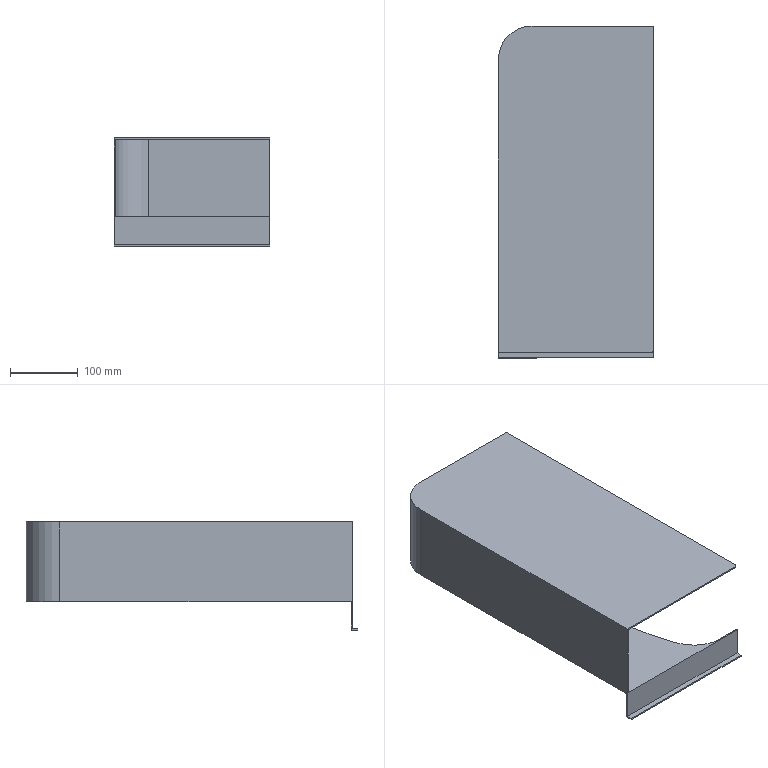Component | SolidWorks | AA-1_B-1 | 1 solid | 22 faces | box 230 x 491 x 160 mm | volume 563290 mm3 | plane 15 | cylinder 7 | commonest cylinder face diameters 120 x2 10 x2 100 x1 96 x1 948.312 x1
build123d program:
from build123d import *

# Parameters (mm, degrees)
SKETCH1_W           = 118
SKETCH1_H           = 483
BOSS_EXTRUDE1_DEPTH = 85
FILLET3_R           = 50
SHELL1_T            = -2
SKETCH3_W           = 170
SKETCH3_H           = 2
BOSS_EXTRUDE3_DEPTH = 40
SKETCH4_W           = 2
SKETCH4_H           = 170
BOSS_EXTRUDE4_DEPTH = 10
BOSS_EXTRUDE7_DEPTH = 30
BOSS_EXTRUDE8_DEPTH = 30
CUT_EXTRUDE7_DEPTH  = 2
CUT_EXTRUDE8_DEPTH  = 2
FILLET2_R           = 5
FILLET4_R           = 5


with BuildPart() as part:
    # Sketch1 → Boss-Extrude1 (new, symmetric)
    with BuildSketch(Plane.XY):
        Rectangle(SKETCH1_W, SKETCH1_H)
    extrude(amount=BOSS_EXTRUDE1_DEPTH, both=True)

    # Fillet3
    fillet3_edges = [part.edges().sort_by_distance(p)[0] for p in [
        (0, 241.5, 85),
    ]]
    fillet(fillet3_edges, radius=FILLET3_R)

    # Shell1
    shell1_openings = [part.faces().sort_by_distance(p)[0] for p in [
        (0, 0, -85),
        (0, -241.5, 0),
    ]]
    offset(amount=SHELL1_T, openings=shell1_openings, kind=Kind.INTERSECTION)

    # Sketch3 → Boss-Extrude3 (add)
    with BuildSketch(Plane(origin=(59, 0, 0), x_dir=(0, 0, -1), z_dir=(1, 0, 0))):
        with Locations((0, -240.5)):
            Rectangle(SKETCH3_W, SKETCH3_H)
    extrude(amount=BOSS_EXTRUDE3_DEPTH)

    # Sketch4 → Boss-Extrude4 (add)
    with BuildSketch(Plane(origin=(0, -239.5, 0), x_dir=(1, 0, 0), z_dir=(0, 1, 0))):
        with Locations((100, 0)):
            Rectangle(SKETCH4_W, SKETCH4_H)
    extrude(amount=-BOSS_EXTRUDE4_DEPTH)

    # Sketch11 → Boss-Extrude7 (add)
    with BuildSketch(Plane(origin=(0, 0, -85), x_dir=(-1, 0, 0), z_dir=(0, 0, -1))):
        Polygon((-101, -239.5), (-101, -249.5), (-99, -249.5), (-99, -241.5), (-57, -241.5), (-57, 239.5), (57, 239.5), (57, -241.5), (59, -241.5), (59, 241.5), (-59, 241.5), (-59, -239.5), align=None)
    extrude(amount=BOSS_EXTRUDE7_DEPTH)

    # Sketch15 → Boss-Extrude8 (add)
    with BuildSketch(Plane(origin=(0, 0, -115), x_dir=(-1, 0, 0), z_dir=(0, 0, -1))):
        Polygon((-101, -239.5), (-101, -249.5), (-99, -249.5), (-99, -241.5), (-57, -241.5), (-57, 239.5), (57, 239.5), (57, -241.5), (59, -241.5), (59, 241.5), (-59, 241.5), (-59, -239.5), align=None)
    extrude(amount=BOSS_EXTRUDE8_DEPTH)

    # Sketch19 → Cut-Extrude7 (cut)
    with BuildSketch(Plane(origin=(59, 0, 0), x_dir=(0, 0, -1), z_dir=(1, 0, 0))):
        with BuildLine():
            Line((154.132, -8.309), (170.602, -162.232))
            Line((170.602, -162.232), (173.325, -174.123))
            ThreePointArc((173.325, -174.123), (163.493, -215.096), (129.143, -239.5))
            Line((129.143, -239.5), (98.418, -239.5))
            ThreePointArc((98.418, -239.5), (72.821, -225.344), (56.958, -200.768))
            ThreePointArc((56.958, -200.768), (34.535, -98.949), (34.907, 5.309))
            ThreePointArc((34.907, 5.309), (101.328, 58.112), (154.132, -8.309))
        make_face()
    extrude(amount=-CUT_EXTRUDE7_DEPTH, mode=Mode.SUBTRACT)

    # Sketch20 → Cut-Extrude8 (cut)
    with BuildSketch(Plane(origin=(59, 0, 0), x_dir=(0, 0, -1), z_dir=(1, 0, 0))):
        with BuildLine():
            Line((145, -239.5), (145, -232.738))
            ThreePointArc((145, -232.738), (137.315, -236.691), (129.143, -239.5))
            Line((129.143, -239.5), (145, -239.5))
        make_face()
    extrude(amount=-CUT_EXTRUDE8_DEPTH, mode=Mode.SUBTRACT)

    # Fillet2
    fillet2_edges = [part.edges().sort_by_distance(p)[0] for p in [
        (58, 30.93, -145),
    ]]
    fillet(fillet2_edges, radius=FILLET2_R)

    # Fillet4
    fillet4_edges = [part.edges().sort_by_distance(p)[0] for p in [
        (-58, -241.5, -145),
    ]]
    fillet(fillet4_edges, radius=FILLET4_R)


with BuildPart() as body_2:
    # Mirror1: mirrored copy
    add(part.part.mirror(Plane.ZX))


solid = body_2.part

# Placed as in the assembly
solid = solid.moved(Location((-531.772, 1.734, 1087.5), (180, -90, 0)))
STEP:
#1=COLOUR_RGB('',0.7922,0.8196,0.9333);
#2=FILL_AREA_STYLE_COLOUR('',#1);
#3=FILL_AREA_STYLE('',(#2));
#4=SURFACE_STYLE_FILL_AREA(#3);
#5=SURFACE_SIDE_STYLE('',(#4));
#6=SURFACE_STYLE_USAGE(.BOTH.,#5);
#7=PRESENTATION_STYLE_ASSIGNMENT((#6));
#8=CARTESIAN_POINT('',(-15.227,9.497,45.059));
#9=VERTEX_POINT('',#8);
#10=CARTESIAN_POINT('',(-15.227,-9.243,45.059));
#11=VERTEX_POINT('',#10);
#12=CARTESIAN_POINT('',(-15.227,9.497,45.059));
#13=DIRECTION('',(0.,-1.,0.));
#14=VECTOR('',#13,39.37);
#15=LINE('',#12,#14);
#16=EDGE_CURVE('',#9,#11,#15,.T.);
#17=ORIENTED_EDGE('',*,*,#16,.F.);
#18=CARTESIAN_POINT('',(-15.227,9.497,40.571));
#19=VERTEX_POINT('',#18);
#20=CARTESIAN_POINT('',(-15.227,9.497,40.571));
#21=DIRECTION('',(0.,0.,1.));
#22=VECTOR('',#21,39.37);
#23=LINE('',#20,#22);
#24=EDGE_CURVE('',#19,#9,#23,.T.);
#25=ORIENTED_EDGE('',*,*,#24,.F.);
#26=CARTESIAN_POINT('',(-15.227,1.837,40.571));
#27=VERTEX_POINT('',#26);
#28=CARTESIAN_POINT('',(-15.227,-9.44,40.571));
#29=DIRECTION('',(-0.,1.,-0.));
#30=VECTOR('',#29,39.37);
#31=LINE('',#28,#30);
#32=EDGE_CURVE('',#27,#19,#31,.T.);
#33=ORIENTED_EDGE('',*,*,#32,.F.);
#34=CARTESIAN_POINT('',(-15.227,1.837,40.492));
#35=VERTEX_POINT('',#34);
#36=CARTESIAN_POINT('',(-15.227,1.837,40.571));
#37=DIRECTION('',(0.,0.,1.));
#38=VECTOR('',#37,39.37);
#39=LINE('',#36,#38);
#40=EDGE_CURVE('',#35,#27,#39,.T.);
#41=ORIENTED_EDGE('',*,*,#40,.F.);
#42=CARTESIAN_POINT('',(-15.227,9.576,40.492));
#43=VERTEX_POINT('',#42);
#44=CARTESIAN_POINT('',(-15.227,9.576,40.492));
#45=DIRECTION('',(0.,-1.,0.));
#46=VECTOR('',#45,39.37);
#47=LINE('',#44,#46);
#48=EDGE_CURVE('',#43,#35,#47,.T.);
#49=ORIENTED_EDGE('',*,*,#48,.F.);
#50=CARTESIAN_POINT('',(-15.227,9.576,45.138));
#51=VERTEX_POINT('',#50);
#52=CARTESIAN_POINT('',(-15.227,9.576,45.138));
#53=DIRECTION('',(-0.,-0.,-1.));
#54=VECTOR('',#53,39.37);
#55=LINE('',#52,#54);
#56=EDGE_CURVE('',#51,#43,#55,.T.);
#57=ORIENTED_EDGE('',*,*,#56,.F.);
#58=CARTESIAN_POINT('',(-15.227,-9.243,45.138));
#59=VERTEX_POINT('',#58);
#60=CARTESIAN_POINT('',(-15.227,-9.44,45.138));
#61=DIRECTION('',(-0.,1.,-0.));
#62=VECTOR('',#61,39.37);
#63=LINE('',#60,#62);
#64=EDGE_CURVE('',#59,#51,#63,.T.);
#65=ORIENTED_EDGE('',*,*,#64,.F.);
#66=CARTESIAN_POINT('',(-15.227,-9.243,45.138));
#67=DIRECTION('',(0.,0.,1.));
#68=VECTOR('',#67,39.37);
#69=LINE('',#66,#68);
#70=EDGE_CURVE('',#11,#59,#69,.T.);
#71=ORIENTED_EDGE('',*,*,#70,.F.);
#72=EDGE_LOOP('',(#17,#25,#33,#41,#49,#57,#65,#71));
#73=FACE_OUTER_BOUND('',#72,.T.);
#74=CARTESIAN_POINT('',(-15.227,0.06827,42.815));
#75=DIRECTION('',(1.,0.,-0.));
#76=DIRECTION('',(0.,0.,1.));
#77=AXIS2_PLACEMENT_3D('',#74,#75,#76);
#78=PLANE('',#77);
#79=ADVANCED_FACE('',(#73),#78,.T.);
#80=CARTESIAN_POINT('',(-15.562,1.697,40.492));
#81=VERTEX_POINT('',#80);
#82=CARTESIAN_POINT('',(-19.562,0.2773,40.492));
#83=VERTEX_POINT('',#82);
#84=CARTESIAN_POINT('',(-17.215,0.009216,40.492));
#85=DIRECTION('',(0.,0.,1.));
#86=DIRECTION('',(1.,0.,0.));
#87=AXIS2_PLACEMENT_3D('',#84,#85,#86);
#88=CIRCLE('',#87,2.362);
#89=EDGE_CURVE('',#81,#83,#88,.T.);
#90=ORIENTED_EDGE('',*,*,#89,.T.);
#91=CARTESIAN_POINT('',(-18.693,-7.836,40.492));
#92=VERTEX_POINT('',#91);
#93=CARTESIAN_POINT('',(-1.015,-1.841,40.492));
#94=DIRECTION('',(0.,0.,1.));
#95=DIRECTION('',(1.,0.,-0.));
#96=AXIS2_PLACEMENT_3D('',#93,#94,#95);
#97=CIRCLE('',#96,18.668);
#98=EDGE_CURVE('',#83,#92,#97,.T.);
#99=ORIENTED_EDGE('',*,*,#98,.T.);
#100=CARTESIAN_POINT('',(-17.061,-9.361,40.492));
#101=VERTEX_POINT('',#100);
#102=CARTESIAN_POINT('',(-16.456,-7.077,40.492));
#103=DIRECTION('',(0.,0.,1.));
#104=DIRECTION('',(1.,0.,0.));
#105=AXIS2_PLACEMENT_3D('',#102,#103,#104);
#106=CIRCLE('',#105,2.362);
#107=EDGE_CURVE('',#92,#101,#106,.T.);
#108=ORIENTED_EDGE('',*,*,#107,.T.);
#109=CARTESIAN_POINT('',(-24.282,-9.361,40.492));
#110=VERTEX_POINT('',#109);
#111=CARTESIAN_POINT('',(-24.282,-9.361,40.492));
#112=DIRECTION('',(-1.,-0.,0.));
#113=VECTOR('',#112,39.37);
#114=LINE('',#111,#113);
#115=EDGE_CURVE('',#101,#110,#114,.T.);
#116=ORIENTED_EDGE('',*,*,#115,.T.);
#117=CARTESIAN_POINT('',(-24.282,7.608,40.492));
#118=VERTEX_POINT('',#117);
#119=CARTESIAN_POINT('',(-24.282,-9.44,40.492));
#120=DIRECTION('',(-0.,1.,-0.));
#121=VECTOR('',#120,39.37);
#122=LINE('',#119,#121);
#123=EDGE_CURVE('',#110,#118,#122,.T.);
#124=ORIENTED_EDGE('',*,*,#123,.T.);
#125=CARTESIAN_POINT('',(-22.314,9.576,40.492));
#126=VERTEX_POINT('',#125);
#127=CARTESIAN_POINT('',(-22.314,7.608,40.492));
#128=DIRECTION('',(0.,0.,1.));
#129=DIRECTION('',(-1.,-0.,0.));
#130=AXIS2_PLACEMENT_3D('',#127,#128,#129);
#131=CIRCLE('',#130,1.969);
#132=EDGE_CURVE('',#126,#118,#131,.T.);
#133=ORIENTED_EDGE('',*,*,#132,.F.);
#134=CARTESIAN_POINT('',(-24.282,9.576,40.492));
#135=DIRECTION('',(1.,0.,-0.));
#136=VECTOR('',#135,39.37);
#137=LINE('',#134,#136);
#138=EDGE_CURVE('',#126,#43,#137,.T.);
#139=ORIENTED_EDGE('',*,*,#138,.T.);
#140=ORIENTED_EDGE('',*,*,#48,.T.);
#141=CARTESIAN_POINT('',(-15.424,1.837,40.492));
#142=DIRECTION('',(0.,0.,1.));
#143=DIRECTION('',(-1.,0.,0.));
#144=AXIS2_PLACEMENT_3D('',#141,#142,#143);
#145=CIRCLE('',#144,0.1969);
#146=EDGE_CURVE('',#81,#35,#145,.T.);
#147=ORIENTED_EDGE('',*,*,#146,.F.);
#148=EDGE_LOOP('',(#90,#99,#108,#116,#124,#133,#139,#140,#147));
#149=FACE_OUTER_BOUND('',#148,.T.);
#150=CARTESIAN_POINT('',(-24.282,-9.44,40.492));
#151=DIRECTION('',(0.,0.,1.));
#152=DIRECTION('',(-1.,-0.,0.));
#153=AXIS2_PLACEMENT_3D('',#150,#151,#152);
#154=PLANE('',#153);
#155=ADVANCED_FACE('',(#149),#154,.F.);
#156=ORIENTED_EDGE('',*,*,#64,.T.);
#157=CARTESIAN_POINT('',(-22.314,9.576,45.138));
#158=VERTEX_POINT('',#157);
#159=CARTESIAN_POINT('',(-24.282,9.576,45.138));
#160=DIRECTION('',(1.,0.,-0.));
#161=VECTOR('',#160,39.37);
#162=LINE('',#159,#161);
#163=EDGE_CURVE('',#158,#51,#162,.T.);
#164=ORIENTED_EDGE('',*,*,#163,.F.);
#165=CARTESIAN_POINT('',(-24.282,7.608,45.138));
#166=VERTEX_POINT('',#165);
#167=CARTESIAN_POINT('',(-22.314,7.608,45.138));
#168=DIRECTION('',(-0.,-0.,-1.));
#169=DIRECTION('',(1.,0.,0.));
#170=AXIS2_PLACEMENT_3D('',#167,#168,#169);
#171=CIRCLE('',#170,1.969);
#172=EDGE_CURVE('',#166,#158,#171,.T.);
#173=ORIENTED_EDGE('',*,*,#172,.F.);
#174=CARTESIAN_POINT('',(-24.282,-9.44,45.138));
#175=VERTEX_POINT('',#174);
#176=CARTESIAN_POINT('',(-24.282,-9.44,45.138));
#177=DIRECTION('',(0.,-1.,0.));
#178=VECTOR('',#177,39.37);
#179=LINE('',#176,#178);
#180=EDGE_CURVE('',#166,#175,#179,.T.);
#181=ORIENTED_EDGE('',*,*,#180,.T.);
#182=CARTESIAN_POINT('',(-15.424,-9.44,45.138));
#183=VERTEX_POINT('',#182);
#184=CARTESIAN_POINT('',(-24.282,-9.44,45.138));
#185=DIRECTION('',(1.,0.,-0.));
#186=VECTOR('',#185,39.37);
#187=LINE('',#184,#186);
#188=EDGE_CURVE('',#175,#183,#187,.T.);
#189=ORIENTED_EDGE('',*,*,#188,.T.);
#190=CARTESIAN_POINT('',(-15.424,-9.243,45.138));
#191=DIRECTION('',(-0.,-0.,-1.));
#192=DIRECTION('',(1.,0.,0.));
#193=AXIS2_PLACEMENT_3D('',#190,#191,#192);
#194=CIRCLE('',#193,0.1969);
#195=EDGE_CURVE('',#59,#183,#194,.T.);
#196=ORIENTED_EDGE('',*,*,#195,.F.);
#197=EDGE_LOOP('',(#156,#164,#173,#181,#189,#196));
#198=FACE_OUTER_BOUND('',#197,.T.);
#199=CARTESIAN_POINT('',(-24.282,-9.44,45.138));
#200=DIRECTION('',(-0.,-0.,-1.));
#201=DIRECTION('',(1.,0.,-0.));
#202=AXIS2_PLACEMENT_3D('',#199,#200,#201);
#203=PLANE('',#202);
#204=ADVANCED_FACE('',(#198),#203,.F.);
#205=ORIENTED_EDGE('',*,*,#188,.F.);
#206=CARTESIAN_POINT('',(-24.282,-9.44,38.917));
#207=VERTEX_POINT('',#206);
#208=CARTESIAN_POINT('',(-24.282,-9.44,40.492));
#209=DIRECTION('',(-0.,-0.,-1.));
#210=VECTOR('',#209,39.37);
#211=LINE('',#208,#210);
#212=EDGE_CURVE('',#175,#207,#211,.T.);
#213=ORIENTED_EDGE('',*,*,#212,.T.);
#214=CARTESIAN_POINT('',(-15.227,-9.44,38.917));
#215=VERTEX_POINT('',#214);
#216=CARTESIAN_POINT('',(-24.282,-9.44,38.917));
#217=DIRECTION('',(1.,0.,-0.));
#218=VECTOR('',#217,39.37);
#219=LINE('',#216,#218);
#220=EDGE_CURVE('',#207,#215,#219,.T.);
#221=ORIENTED_EDGE('',*,*,#220,.T.);
#222=CARTESIAN_POINT('',(-15.227,-9.44,40.571));
#223=VERTEX_POINT('',#222);
#224=CARTESIAN_POINT('',(-15.227,-9.44,38.917));
#225=DIRECTION('',(0.,0.,1.));
#226=VECTOR('',#225,39.37);
#227=LINE('',#224,#226);
#228=EDGE_CURVE('',#215,#223,#227,.T.);
#229=ORIENTED_EDGE('',*,*,#228,.T.);
#230=CARTESIAN_POINT('',(-24.204,-9.44,40.571));
#231=VERTEX_POINT('',#230);
#232=CARTESIAN_POINT('',(-24.282,-9.44,40.571));
#233=DIRECTION('',(1.,0.,-0.));
#234=VECTOR('',#233,39.37);
#235=LINE('',#232,#234);
#236=EDGE_CURVE('',#231,#223,#235,.T.);
#237=ORIENTED_EDGE('',*,*,#236,.F.);
#238=CARTESIAN_POINT('',(-24.204,-9.44,45.059));
#239=VERTEX_POINT('',#238);
#240=CARTESIAN_POINT('',(-24.204,-9.44,40.492));
#241=DIRECTION('',(-0.,-0.,-1.));
#242=VECTOR('',#241,39.37);
#243=LINE('',#240,#242);
#244=EDGE_CURVE('',#239,#231,#243,.T.);
#245=ORIENTED_EDGE('',*,*,#244,.F.);
#246=CARTESIAN_POINT('',(-15.424,-9.44,45.059));
#247=VERTEX_POINT('',#246);
#248=CARTESIAN_POINT('',(-24.282,-9.44,45.059));
#249=DIRECTION('',(1.,0.,-0.));
#250=VECTOR('',#249,39.37);
#251=LINE('',#248,#250);
#252=EDGE_CURVE('',#239,#247,#251,.T.);
#253=ORIENTED_EDGE('',*,*,#252,.T.);
#254=CARTESIAN_POINT('',(-15.424,-9.44,45.059));
#255=DIRECTION('',(-0.,-0.,-1.));
#256=VECTOR('',#255,39.37);
#257=LINE('',#254,#256);
#258=EDGE_CURVE('',#183,#247,#257,.T.);
#259=ORIENTED_EDGE('',*,*,#258,.F.);
#260=EDGE_LOOP('',(#205,#213,#221,#229,#237,#245,#253,#259));
#261=FACE_OUTER_BOUND('',#260,.T.);
#262=CARTESIAN_POINT('',(-24.282,-9.44,40.492));
#263=DIRECTION('',(-0.,1.,-0.));
#264=DIRECTION('',(0.,0.,1.));
#265=AXIS2_PLACEMENT_3D('',#262,#263,#264);
#266=PLANE('',#265);
#267=ADVANCED_FACE('',(#261),#266,.F.);
#268=ORIENTED_EDGE('',*,*,#163,.T.);
#269=ORIENTED_EDGE('',*,*,#56,.T.);
#270=ORIENTED_EDGE('',*,*,#138,.F.);
#271=CARTESIAN_POINT('',(-22.314,9.576,40.492));
#272=DIRECTION('',(-0.,-0.,-1.));
#273=VECTOR('',#272,39.37);
#274=LINE('',#271,#273);
#275=EDGE_CURVE('',#158,#126,#274,.T.);
#276=ORIENTED_EDGE('',*,*,#275,.F.);
#277=EDGE_LOOP('',(#268,#269,#270,#276));
#278=FACE_OUTER_BOUND('',#277,.T.);
#279=CARTESIAN_POINT('',(-24.282,9.576,40.492));
#280=DIRECTION('',(0.,-1.,0.));
#281=DIRECTION('',(-0.,-0.,-1.));
#282=AXIS2_PLACEMENT_3D('',#279,#280,#281);
#283=PLANE('',#282);
#284=ADVANCED_FACE('',(#278),#283,.F.);
#285=ORIENTED_EDGE('',*,*,#212,.F.);
#286=ORIENTED_EDGE('',*,*,#180,.F.);
#287=CARTESIAN_POINT('',(-24.282,7.608,45.138));
#288=DIRECTION('',(0.,0.,1.));
#289=VECTOR('',#288,39.37);
#290=LINE('',#287,#289);
#291=EDGE_CURVE('',#118,#166,#290,.T.);
#292=ORIENTED_EDGE('',*,*,#291,.F.);
#293=ORIENTED_EDGE('',*,*,#123,.F.);
#294=CARTESIAN_POINT('',(-24.282,-9.361,38.839));
#295=VERTEX_POINT('',#294);
#296=CARTESIAN_POINT('',(-24.282,-9.361,38.917));
#297=DIRECTION('',(0.,0.,1.));
#298=VECTOR('',#297,39.37);
#299=LINE('',#296,#298);
#300=EDGE_CURVE('',#295,#110,#299,.T.);
#301=ORIENTED_EDGE('',*,*,#300,.F.);
#302=CARTESIAN_POINT('',(-24.282,-9.755,38.839));
#303=VERTEX_POINT('',#302);
#304=CARTESIAN_POINT('',(-24.282,-9.755,38.839));
#305=DIRECTION('',(-0.,1.,-0.));
#306=VECTOR('',#305,39.37);
#307=LINE('',#304,#306);
#308=EDGE_CURVE('',#303,#295,#307,.T.);
#309=ORIENTED_EDGE('',*,*,#308,.F.);
#310=CARTESIAN_POINT('',(-24.282,-9.755,38.917));
#311=VERTEX_POINT('',#310);
#312=CARTESIAN_POINT('',(-24.282,-9.755,38.917));
#313=DIRECTION('',(-0.,-0.,-1.));
#314=VECTOR('',#313,39.37);
#315=LINE('',#312,#314);
#316=EDGE_CURVE('',#311,#303,#315,.T.);
#317=ORIENTED_EDGE('',*,*,#316,.F.);
#318=CARTESIAN_POINT('',(-24.282,-9.755,38.917));
#319=DIRECTION('',(-0.,1.,-0.));
#320=VECTOR('',#319,39.37);
#321=LINE('',#318,#320);
#322=EDGE_CURVE('',#311,#207,#321,.T.);
#323=ORIENTED_EDGE('',*,*,#322,.T.);
#324=EDGE_LOOP('',(#285,#286,#292,#293,#301,#309,#317,#323));
#325=FACE_OUTER_BOUND('',#324,.T.);
#326=CARTESIAN_POINT('',(-24.282,0.06827,42.815));
#327=DIRECTION('',(-1.,-0.,0.));
#328=DIRECTION('',(-0.,-0.,-1.));
#329=AXIS2_PLACEMENT_3D('',#326,#327,#328);
#330=PLANE('',#329);
#331=ADVANCED_FACE('',(#325),#330,.T.);
#332=ORIENTED_EDGE('',*,*,#132,.T.);
#333=ORIENTED_EDGE('',*,*,#291,.T.);
#334=ORIENTED_EDGE('',*,*,#172,.T.);
#335=ORIENTED_EDGE('',*,*,#275,.T.);
#336=EDGE_LOOP('',(#332,#333,#334,#335));
#337=FACE_OUTER_BOUND('',#336,.T.);
#338=CARTESIAN_POINT('',(-22.314,7.608,42.815));
#339=DIRECTION('',(-0.,-0.,-1.));
#340=DIRECTION('',(0.,1.,0.));
#341=AXIS2_PLACEMENT_3D('',#338,#339,#340);
#342=CYLINDRICAL_SURFACE('',#341,1.969);
#343=ADVANCED_FACE('',(#337),#342,.T.);
#344=ORIENTED_EDGE('',*,*,#252,.F.);
#345=CARTESIAN_POINT('',(-24.204,7.608,45.059));
#346=VERTEX_POINT('',#345);
#347=CARTESIAN_POINT('',(-24.204,-9.44,45.059));
#348=DIRECTION('',(0.,-1.,0.));
#349=VECTOR('',#348,39.37);
#350=LINE('',#347,#349);
#351=EDGE_CURVE('',#346,#239,#350,.T.);
#352=ORIENTED_EDGE('',*,*,#351,.F.);
#353=CARTESIAN_POINT('',(-22.314,9.497,45.059));
#354=VERTEX_POINT('',#353);
#355=CARTESIAN_POINT('',(-22.314,7.608,45.059));
#356=DIRECTION('',(-0.,-0.,-1.));
#357=DIRECTION('',(1.,0.,0.));
#358=AXIS2_PLACEMENT_3D('',#355,#356,#357);
#359=CIRCLE('',#358,1.89);
#360=EDGE_CURVE('',#346,#354,#359,.T.);
#361=ORIENTED_EDGE('',*,*,#360,.T.);
#362=CARTESIAN_POINT('',(-24.282,9.497,45.059));
#363=DIRECTION('',(1.,0.,-0.));
#364=VECTOR('',#363,39.37);
#365=LINE('',#362,#364);
#366=EDGE_CURVE('',#354,#9,#365,.T.);
#367=ORIENTED_EDGE('',*,*,#366,.T.);
#368=ORIENTED_EDGE('',*,*,#16,.T.);
#369=CARTESIAN_POINT('',(-15.424,-9.243,45.059));
#370=DIRECTION('',(0.,0.,1.));
#371=DIRECTION('',(1.,0.,0.));
#372=AXIS2_PLACEMENT_3D('',#369,#370,#371);
#373=CIRCLE('',#372,0.1969);
#374=EDGE_CURVE('',#247,#11,#373,.T.);
#375=ORIENTED_EDGE('',*,*,#374,.F.);
#376=EDGE_LOOP('',(#344,#352,#361,#367,#368,#375));
#377=FACE_OUTER_BOUND('',#376,.T.);
#378=CARTESIAN_POINT('',(-24.282,-9.44,45.059));
#379=DIRECTION('',(-0.,-0.,-1.));
#380=DIRECTION('',(1.,0.,-0.));
#381=AXIS2_PLACEMENT_3D('',#378,#379,#380);
#382=PLANE('',#381);
#383=ADVANCED_FACE('',(#377),#382,.T.);
#384=ORIENTED_EDGE('',*,*,#32,.T.);
#385=CARTESIAN_POINT('',(-22.314,9.497,40.571));
#386=VERTEX_POINT('',#385);
#387=CARTESIAN_POINT('',(-24.282,9.497,40.571));
#388=DIRECTION('',(1.,0.,-0.));
#389=VECTOR('',#388,39.37);
#390=LINE('',#387,#389);
#391=EDGE_CURVE('',#386,#19,#390,.T.);
#392=ORIENTED_EDGE('',*,*,#391,.F.);
#393=CARTESIAN_POINT('',(-24.204,7.608,40.571));
#394=VERTEX_POINT('',#393);
#395=CARTESIAN_POINT('',(-22.314,7.608,40.571));
#396=DIRECTION('',(0.,0.,1.));
#397=DIRECTION('',(-1.,-0.,0.));
#398=AXIS2_PLACEMENT_3D('',#395,#396,#397);
#399=CIRCLE('',#398,1.89);
#400=EDGE_CURVE('',#386,#394,#399,.T.);
#401=ORIENTED_EDGE('',*,*,#400,.T.);
#402=CARTESIAN_POINT('',(-24.204,-9.44,40.571));
#403=DIRECTION('',(-0.,1.,-0.));
#404=VECTOR('',#403,39.37);
#405=LINE('',#402,#404);
#406=EDGE_CURVE('',#231,#394,#405,.T.);
#407=ORIENTED_EDGE('',*,*,#406,.F.);
#408=ORIENTED_EDGE('',*,*,#236,.T.);
#409=CARTESIAN_POINT('',(-15.227,-9.361,40.571));
#410=VERTEX_POINT('',#409);
#411=CARTESIAN_POINT('',(-15.227,-9.44,40.571));
#412=DIRECTION('',(-0.,1.,-0.));
#413=VECTOR('',#412,39.37);
#414=LINE('',#411,#413);
#415=EDGE_CURVE('',#223,#410,#414,.T.);
#416=ORIENTED_EDGE('',*,*,#415,.T.);
#417=CARTESIAN_POINT('',(-17.061,-9.361,40.571));
#418=VERTEX_POINT('',#417);
#419=CARTESIAN_POINT('',(-17.061,-9.361,40.571));
#420=DIRECTION('',(1.,0.,-0.));
#421=VECTOR('',#420,39.37);
#422=LINE('',#419,#421);
#423=EDGE_CURVE('',#418,#410,#422,.T.);
#424=ORIENTED_EDGE('',*,*,#423,.F.);
#425=CARTESIAN_POINT('',(-18.693,-7.836,40.571));
#426=VERTEX_POINT('',#425);
#427=CARTESIAN_POINT('',(-16.456,-7.077,40.571));
#428=DIRECTION('',(0.,0.,1.));
#429=DIRECTION('',(1.,0.,0.));
#430=AXIS2_PLACEMENT_3D('',#427,#428,#429);
#431=CIRCLE('',#430,2.362);
#432=EDGE_CURVE('',#426,#418,#431,.T.);
#433=ORIENTED_EDGE('',*,*,#432,.F.);
#434=CARTESIAN_POINT('',(-19.562,0.2773,40.571));
#435=VERTEX_POINT('',#434);
#436=CARTESIAN_POINT('',(-1.015,-1.841,40.571));
#437=DIRECTION('',(0.,0.,1.));
#438=DIRECTION('',(1.,0.,-0.));
#439=AXIS2_PLACEMENT_3D('',#436,#437,#438);
#440=CIRCLE('',#439,18.668);
#441=EDGE_CURVE('',#435,#426,#440,.T.);
#442=ORIENTED_EDGE('',*,*,#441,.F.);
#443=CARTESIAN_POINT('',(-15.562,1.697,40.571));
#444=VERTEX_POINT('',#443);
#445=CARTESIAN_POINT('',(-17.215,0.009216,40.571));
#446=DIRECTION('',(0.,0.,1.));
#447=DIRECTION('',(1.,0.,0.));
#448=AXIS2_PLACEMENT_3D('',#445,#446,#447);
#449=CIRCLE('',#448,2.362);
#450=EDGE_CURVE('',#444,#435,#449,.T.);
#451=ORIENTED_EDGE('',*,*,#450,.F.);
#452=CARTESIAN_POINT('',(-15.424,1.837,40.571));
#453=DIRECTION('',(-0.,-0.,-1.));
#454=DIRECTION('',(-1.,0.,0.));
#455=AXIS2_PLACEMENT_3D('',#452,#453,#454);
#456=CIRCLE('',#455,0.1969);
#457=EDGE_CURVE('',#27,#444,#456,.T.);
#458=ORIENTED_EDGE('',*,*,#457,.F.);
#459=EDGE_LOOP('',(#384,#392,#401,#407,#408,#416,#424,#433,#442,#451,#458));
#460=FACE_OUTER_BOUND('',#459,.T.);
#461=CARTESIAN_POINT('',(-24.282,-9.44,40.571));
#462=DIRECTION('',(0.,0.,1.));
#463=DIRECTION('',(-1.,-0.,0.));
#464=AXIS2_PLACEMENT_3D('',#461,#462,#463);
#465=PLANE('',#464);
#466=ADVANCED_FACE('',(#460),#465,.T.);
#467=ORIENTED_EDGE('',*,*,#366,.F.);
#468=CARTESIAN_POINT('',(-22.314,9.497,40.492));
#469=DIRECTION('',(-0.,-0.,-1.));
#470=VECTOR('',#469,39.37);
#471=LINE('',#468,#470);
#472=EDGE_CURVE('',#354,#386,#471,.T.);
#473=ORIENTED_EDGE('',*,*,#472,.T.);
#474=ORIENTED_EDGE('',*,*,#391,.T.);
#475=ORIENTED_EDGE('',*,*,#24,.T.);
#476=EDGE_LOOP('',(#467,#473,#474,#475));
#477=FACE_OUTER_BOUND('',#476,.T.);
#478=CARTESIAN_POINT('',(-24.282,9.497,40.492));
#479=DIRECTION('',(0.,-1.,0.));
#480=DIRECTION('',(-0.,-0.,-1.));
#481=AXIS2_PLACEMENT_3D('',#478,#479,#480);
#482=PLANE('',#481);
#483=ADVANCED_FACE('',(#477),#482,.T.);
#484=ORIENTED_EDGE('',*,*,#406,.T.);
#485=CARTESIAN_POINT('',(-24.204,7.608,42.815));
#486=DIRECTION('',(0.,0.,1.));
#487=VECTOR('',#486,39.37);
#488=LINE('',#485,#487);
#489=EDGE_CURVE('',#394,#346,#488,.T.);
#490=ORIENTED_EDGE('',*,*,#489,.T.);
#491=ORIENTED_EDGE('',*,*,#351,.T.);
#492=ORIENTED_EDGE('',*,*,#244,.T.);
#493=EDGE_LOOP('',(#484,#490,#491,#492));
#494=FACE_OUTER_BOUND('',#493,.T.);
#495=CARTESIAN_POINT('',(-24.204,0.06827,42.815));
#496=DIRECTION('',(-1.,-0.,0.));
#497=DIRECTION('',(-0.,-0.,-1.));
#498=AXIS2_PLACEMENT_3D('',#495,#496,#497);
#499=PLANE('',#498);
#500=ADVANCED_FACE('',(#494),#499,.F.);
#501=ORIENTED_EDGE('',*,*,#400,.F.);
#502=ORIENTED_EDGE('',*,*,#472,.F.);
#503=ORIENTED_EDGE('',*,*,#360,.F.);
#504=ORIENTED_EDGE('',*,*,#489,.F.);
#505=EDGE_LOOP('',(#501,#502,#503,#504));
#506=FACE_OUTER_BOUND('',#505,.T.);
#507=CARTESIAN_POINT('',(-22.314,7.608,42.815));
#508=DIRECTION('',(-0.,-0.,-1.));
#509=DIRECTION('',(0.,1.,0.));
#510=AXIS2_PLACEMENT_3D('',#507,#508,#509);
#511=CYLINDRICAL_SURFACE('',#510,1.89);
#512=ADVANCED_FACE('',(#506),#511,.F.);
#513=CARTESIAN_POINT('',(-15.227,-9.361,38.839));
#514=VERTEX_POINT('',#513);
#515=CARTESIAN_POINT('',(-15.227,-9.361,40.492));
#516=DIRECTION('',(-0.,-0.,-1.));
#517=VECTOR('',#516,39.37);
#518=LINE('',#515,#517);
#519=EDGE_CURVE('',#410,#514,#518,.T.);
#520=ORIENTED_EDGE('',*,*,#519,.T.);
#521=CARTESIAN_POINT('',(-17.589,-9.361,38.839));
#522=DIRECTION('',(1.,0.,-0.));
#523=VECTOR('',#522,39.37);
#524=LINE('',#521,#523);
#525=EDGE_CURVE('',#295,#514,#524,.T.);
#526=ORIENTED_EDGE('',*,*,#525,.F.);
#527=ORIENTED_EDGE('',*,*,#300,.T.);
#528=ORIENTED_EDGE('',*,*,#115,.F.);
#529=CARTESIAN_POINT('',(-17.061,-9.361,40.571));
#530=DIRECTION('',(-0.,-0.,-1.));
#531=VECTOR('',#530,39.37);
#532=LINE('',#529,#531);
#533=EDGE_CURVE('',#418,#101,#532,.T.);
#534=ORIENTED_EDGE('',*,*,#533,.F.);
#535=ORIENTED_EDGE('',*,*,#423,.T.);
#536=EDGE_LOOP('',(#520,#526,#527,#528,#534,#535));
#537=FACE_OUTER_BOUND('',#536,.T.);
#538=CARTESIAN_POINT('',(-24.282,-9.361,38.917));
#539=DIRECTION('',(0.,-1.,0.));
#540=DIRECTION('',(1.,0.,-0.));
#541=AXIS2_PLACEMENT_3D('',#538,#539,#540);
#542=PLANE('',#541);
#543=ADVANCED_FACE('',(#537),#542,.F.);
#544=ORIENTED_EDGE('',*,*,#322,.F.);
#545=CARTESIAN_POINT('',(-15.227,-9.755,38.917));
#546=VERTEX_POINT('',#545);
#547=CARTESIAN_POINT('',(-17.589,-9.755,38.917));
#548=DIRECTION('',(-1.,-0.,0.));
#549=VECTOR('',#548,39.37);
#550=LINE('',#547,#549);
#551=EDGE_CURVE('',#546,#311,#550,.T.);
#552=ORIENTED_EDGE('',*,*,#551,.F.);
#553=CARTESIAN_POINT('',(-15.227,-9.755,38.917));
#554=DIRECTION('',(-0.,1.,-0.));
#555=VECTOR('',#554,39.37);
#556=LINE('',#553,#555);
#557=EDGE_CURVE('',#546,#215,#556,.T.);
#558=ORIENTED_EDGE('',*,*,#557,.T.);
#559=ORIENTED_EDGE('',*,*,#220,.F.);
#560=EDGE_LOOP('',(#544,#552,#558,#559));
#561=FACE_OUTER_BOUND('',#560,.T.);
#562=CARTESIAN_POINT('',(-17.589,-9.755,38.917));
#563=DIRECTION('',(0.,0.,1.));
#564=DIRECTION('',(-1.,-0.,0.));
#565=AXIS2_PLACEMENT_3D('',#562,#563,#564);
#566=PLANE('',#565);
#567=ADVANCED_FACE('',(#561),#566,.T.);
#568=ORIENTED_EDGE('',*,*,#525,.T.);
#569=CARTESIAN_POINT('',(-15.227,-9.755,38.839));
#570=VERTEX_POINT('',#569);
#571=CARTESIAN_POINT('',(-15.227,-9.361,38.839));
#572=DIRECTION('',(0.,-1.,0.));
#573=VECTOR('',#572,39.37);
#574=LINE('',#571,#573);
#575=EDGE_CURVE('',#514,#570,#574,.T.);
#576=ORIENTED_EDGE('',*,*,#575,.T.);
#577=CARTESIAN_POINT('',(-17.589,-9.755,38.839));
#578=DIRECTION('',(1.,0.,-0.));
#579=VECTOR('',#578,39.37);
#580=LINE('',#577,#579);
#581=EDGE_CURVE('',#303,#570,#580,.T.);
#582=ORIENTED_EDGE('',*,*,#581,.F.);
#583=ORIENTED_EDGE('',*,*,#308,.T.);
#584=EDGE_LOOP('',(#568,#576,#582,#583));
#585=FACE_OUTER_BOUND('',#584,.T.);
#586=CARTESIAN_POINT('',(-17.589,-9.755,38.839));
#587=DIRECTION('',(-0.,-0.,-1.));
#588=DIRECTION('',(1.,0.,-0.));
#589=AXIS2_PLACEMENT_3D('',#586,#587,#588);
#590=PLANE('',#589);
#591=ADVANCED_FACE('',(#585),#590,.T.);
#592=ORIENTED_EDGE('',*,*,#551,.T.);
#593=ORIENTED_EDGE('',*,*,#316,.T.);
#594=ORIENTED_EDGE('',*,*,#581,.T.);
#595=CARTESIAN_POINT('',(-15.227,-9.755,38.839));
#596=DIRECTION('',(0.,0.,1.));
#597=VECTOR('',#596,39.37);
#598=LINE('',#595,#597);
#599=EDGE_CURVE('',#570,#546,#598,.T.);
#600=ORIENTED_EDGE('',*,*,#599,.T.);
#601=EDGE_LOOP('',(#592,#593,#594,#600));
#602=FACE_OUTER_BOUND('',#601,.T.);
#603=CARTESIAN_POINT('',(-20.936,-9.755,42.815));
#604=DIRECTION('',(-0.,1.,-0.));
#605=DIRECTION('',(-1.,-0.,0.));
#606=AXIS2_PLACEMENT_3D('',#603,#604,#605);
#607=PLANE('',#606);
#608=ADVANCED_FACE('',(#602),#607,.F.);
#609=ORIENTED_EDGE('',*,*,#415,.F.);
#610=ORIENTED_EDGE('',*,*,#228,.F.);
#611=ORIENTED_EDGE('',*,*,#557,.F.);
#612=ORIENTED_EDGE('',*,*,#599,.F.);
#613=ORIENTED_EDGE('',*,*,#575,.F.);
#614=ORIENTED_EDGE('',*,*,#519,.F.);
#615=EDGE_LOOP('',(#609,#610,#611,#612,#613,#614));
#616=FACE_OUTER_BOUND('',#615,.T.);
#617=CARTESIAN_POINT('',(-15.227,0.06827,42.815));
#618=DIRECTION('',(1.,0.,-0.));
#619=DIRECTION('',(0.,0.,1.));
#620=AXIS2_PLACEMENT_3D('',#617,#618,#619);
#621=PLANE('',#620);
#622=ADVANCED_FACE('',(#616),#621,.T.);
#623=ORIENTED_EDGE('',*,*,#98,.F.);
#624=CARTESIAN_POINT('',(-19.562,0.2773,40.571));
#625=DIRECTION('',(-0.,-0.,-1.));
#626=VECTOR('',#625,39.37);
#627=LINE('',#624,#626);
#628=EDGE_CURVE('',#435,#83,#627,.T.);
#629=ORIENTED_EDGE('',*,*,#628,.F.);
#630=ORIENTED_EDGE('',*,*,#441,.T.);
#631=CARTESIAN_POINT('',(-18.693,-7.836,40.571));
#632=DIRECTION('',(-0.,-0.,-1.));
#633=VECTOR('',#632,39.37);
#634=LINE('',#631,#633);
#635=EDGE_CURVE('',#426,#92,#634,.T.);
#636=ORIENTED_EDGE('',*,*,#635,.T.);
#637=EDGE_LOOP('',(#623,#629,#630,#636));
#638=FACE_OUTER_BOUND('',#637,.T.);
#639=CARTESIAN_POINT('',(-1.015,-1.841,40.571));
#640=DIRECTION('',(-0.,-0.,-1.));
#641=DIRECTION('',(1.,0.,-0.));
#642=AXIS2_PLACEMENT_3D('',#639,#640,#641);
#643=CYLINDRICAL_SURFACE('',#642,18.668);
#644=ADVANCED_FACE('',(#638),#643,.F.);
#645=ORIENTED_EDGE('',*,*,#450,.T.);
#646=ORIENTED_EDGE('',*,*,#628,.T.);
#647=ORIENTED_EDGE('',*,*,#89,.F.);
#648=CARTESIAN_POINT('',(-15.562,1.697,40.571));
#649=DIRECTION('',(-0.,-0.,-1.));
#650=VECTOR('',#649,39.37);
#651=LINE('',#648,#650);
#652=EDGE_CURVE('',#444,#81,#651,.T.);
#653=ORIENTED_EDGE('',*,*,#652,.F.);
#654=EDGE_LOOP('',(#645,#646,#647,#653));
#655=FACE_OUTER_BOUND('',#654,.T.);
#656=CARTESIAN_POINT('',(-17.215,0.009216,40.571));
#657=DIRECTION('',(-0.,-0.,-1.));
#658=DIRECTION('',(1.,0.,0.));
#659=AXIS2_PLACEMENT_3D('',#656,#657,#658);
#660=CYLINDRICAL_SURFACE('',#659,2.362);
#661=ADVANCED_FACE('',(#655),#660,.F.);
#662=ORIENTED_EDGE('',*,*,#107,.F.);
#663=ORIENTED_EDGE('',*,*,#635,.F.);
#664=ORIENTED_EDGE('',*,*,#432,.T.);
#665=ORIENTED_EDGE('',*,*,#533,.T.);
#666=EDGE_LOOP('',(#662,#663,#664,#665));
#667=FACE_OUTER_BOUND('',#666,.T.);
#668=CARTESIAN_POINT('',(-16.456,-7.077,40.571));
#669=DIRECTION('',(-0.,-0.,-1.));
#670=DIRECTION('',(1.,0.,0.));
#671=AXIS2_PLACEMENT_3D('',#668,#669,#670);
#672=CYLINDRICAL_SURFACE('',#671,2.362);
#673=ADVANCED_FACE('',(#667),#672,.F.);
#674=ORIENTED_EDGE('',*,*,#457,.T.);
#675=ORIENTED_EDGE('',*,*,#652,.T.);
#676=ORIENTED_EDGE('',*,*,#146,.T.);
#677=ORIENTED_EDGE('',*,*,#40,.T.);
#678=EDGE_LOOP('',(#674,#675,#676,#677));
#679=FACE_OUTER_BOUND('',#678,.T.);
#680=CARTESIAN_POINT('',(-15.424,1.837,40.571));
#681=DIRECTION('',(-0.,-0.,-1.));
#682=DIRECTION('',(1.,0.,0.));
#683=AXIS2_PLACEMENT_3D('',#680,#681,#682);
#684=CYLINDRICAL_SURFACE('',#683,0.1969);
#685=ADVANCED_FACE('',(#679),#684,.T.);
#686=ORIENTED_EDGE('',*,*,#374,.T.);
#687=ORIENTED_EDGE('',*,*,#70,.T.);
#688=ORIENTED_EDGE('',*,*,#195,.T.);
#689=ORIENTED_EDGE('',*,*,#258,.T.);
#690=EDGE_LOOP('',(#686,#687,#688,#689));
#691=FACE_OUTER_BOUND('',#690,.T.);
#692=CARTESIAN_POINT('',(-15.424,-9.243,42.815));
#693=DIRECTION('',(-0.,-0.,-1.));
#694=DIRECTION('',(0.,1.,0.));
#695=AXIS2_PLACEMENT_3D('',#692,#693,#694);
#696=CYLINDRICAL_SURFACE('',#695,0.1969);
#697=ADVANCED_FACE('',(#691),#696,.T.);
#698=CLOSED_SHELL('',(#79,#155,#204,#267,#284,#331,#343,#383,#466,#483,#500,#512,#543,#567,#591,#608,#622,#644,#661,#673,#685,#697));
#699=MANIFOLD_SOLID_BREP('',#698);
#700=STYLED_ITEM('',(#7),#699);
#701=PRESENTATION_LAYER_ASSIGNMENT('','',(#700));
#702=CARTESIAN_POINT('',(0.,0.,0.));
#703=DIRECTION('',(0.,0.,1.));
#704=DIRECTION('',(1.,0.,0.));
#705=AXIS2_PLACEMENT_3D('',#702,#703,#704);
#706=(LENGTH_UNIT()NAMED_UNIT(*)SI_UNIT($,.METRE.));
#707=LENGTH_MEASURE_WITH_UNIT(LENGTH_MEASURE(0.0254),#706);
#708=DIMENSIONAL_EXPONENTS(1.,0.,0.,0.,0.,0.,0.);
#709=(CONVERSION_BASED_UNIT('',#707)LENGTH_UNIT()NAMED_UNIT(#708));
#710=UNCERTAINTY_MEASURE_WITH_UNIT(LENGTH_MEASURE(0.00001),#709,'','');
#711=(NAMED_UNIT(*)PLANE_ANGLE_UNIT()SI_UNIT($,.RADIAN.));
#712=(NAMED_UNIT(*)SI_UNIT($,.STERADIAN.)SOLID_ANGLE_UNIT());
#713=(GEOMETRIC_REPRESENTATION_CONTEXT(3)GLOBAL_UNCERTAINTY_ASSIGNED_CONTEXT((#710))GLOBAL_UNIT_ASSIGNED_CONTEXT((#709,#711,#712))REPRESENTATION_CONTEXT('',''));
#714=ADVANCED_BREP_SHAPE_REPRESENTATION('',(#699,#705),#713);
#715=(LENGTH_UNIT()NAMED_UNIT(*)SI_UNIT($,.METRE.));
#716=LENGTH_MEASURE_WITH_UNIT(LENGTH_MEASURE(0.0254),#715);
#717=DIMENSIONAL_EXPONENTS(1.,0.,0.,0.,0.,0.,0.);
#718=(CONVERSION_BASED_UNIT('',#716)LENGTH_UNIT()NAMED_UNIT(#717));
#719=UNCERTAINTY_MEASURE_WITH_UNIT(LENGTH_MEASURE(0.00001),#718,'','');
#720=(NAMED_UNIT(*)PLANE_ANGLE_UNIT()SI_UNIT($,.RADIAN.));
#721=(NAMED_UNIT(*)SI_UNIT($,.STERADIAN.)SOLID_ANGLE_UNIT());
#722=(GEOMETRIC_REPRESENTATION_CONTEXT(3)GLOBAL_UNCERTAINTY_ASSIGNED_CONTEXT((#719))GLOBAL_UNIT_ASSIGNED_CONTEXT((#718,#720,#721))REPRESENTATION_CONTEXT('',''));
#723=MECHANICAL_DESIGN_GEOMETRIC_PRESENTATION_REPRESENTATION('',(#700),#722);